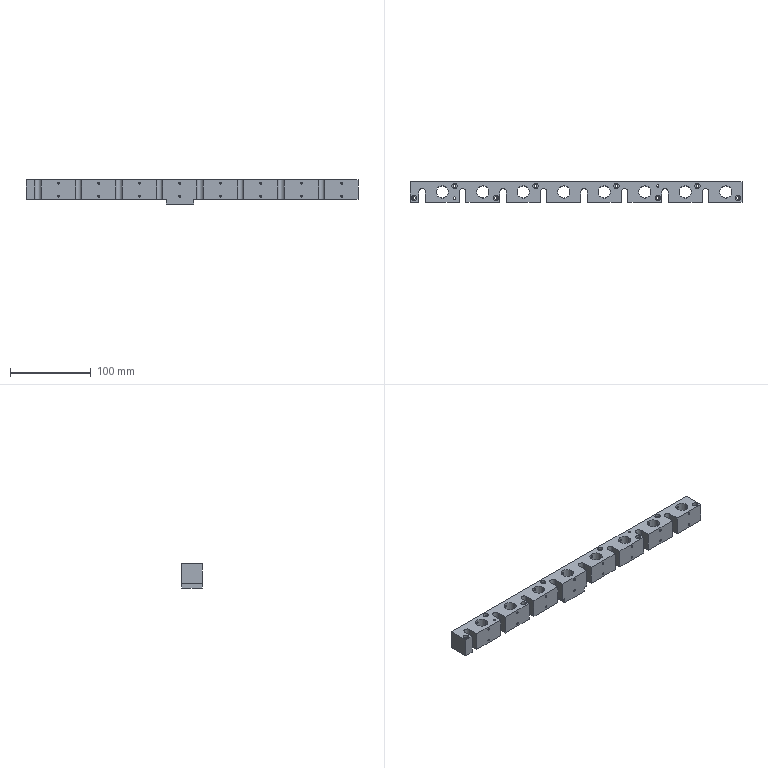Component | SolidWorks | 002MaterialPickingModuleA-1_004SidePlugModule-1_J-009-1 | 1 solid | 174 faces | box 410 x 25 x 30 mm | volume 188018 mm3 | cylinder 128 | plane 42 | cone 4 | commonest cylinder face diameters 2.5 x64 6.5 x16 3.4 x16 15 x16 8.1 x8 3 x4 3.3 x4 | material 45
build123d program:
from build123d import *

# Parameters (mm, degrees)
SKETCH1_W                                       = 440
SKETCH1_H                                       = 24
BOSS_EXTRUDE1_DEPTH                             = 12.5
SKETCH2_R                                       = 7.5
CUT_EXTRUDE1_DEPTH                              = 222.658
CUT_EXTRUDE2_DEPTH                              = 222.658
LPATTERN1_COUNT                                 = 8
LPATTERN1_PITCH                                 = 50
SKETCH4_W                                       = 34
SKETCH4_H                                       = 25
SKETCH4_R                                       = 7.5
BOSS_EXTRUDE2_DEPTH                             = 6
M4_TAPPED_HOLE1_D                               = 3.3
M4_TAPPED_HOLE1_DEPTH                           = 10.1
M4_TAPPED_HOLE1_TIP                             = 0.9914
SKETCH8_W                                       = 30
SKETCH8_H                                       = 25
CUT_EXTRUDE4_DEPTH                              = 223.388
M3_HEX_SOCKET_HEAD_CAP_SCREW_CBORE1_D           = 3.4
M3_HEX_SOCKET_HEAD_CAP_SCREW_CBORE1_CBORE_D     = 6.5
M3_HEX_SOCKET_HEAD_CAP_SCREW_CBORE1_CBORE_DEPTH = 3.4
SIZE_MM_DOWEL_PIN_HOLE1_D                       = 3
M3_TAPPED_HOLE1_D                               = 2.5
LPATTERN2_COUNT                                 = 8
LPATTERN2_PITCH                                 = 50


with BuildPart() as part:
    # Sketch1 → Boss-Extrude1 (new, symmetric)
    with BuildSketch(Plane(origin=(0, 0, 0), x_dir=(1, 0, 0), z_dir=(0, 1, 0))):
        Rectangle(SKETCH1_W, SKETCH1_H)
    extrude(amount=BOSS_EXTRUDE1_DEPTH, both=True)

    # Sketch2 → Cut-Extrude1 (cut, through all)
    with BuildSketch(Plane.XY.offset(12)):
        Circle(SKETCH2_R)
        with Locations((-50, 0)):
            Circle(SKETCH2_R)
        with Locations((-100, 0)):
            Circle(SKETCH2_R)
        with Locations((50, 0)):
            Circle(SKETCH2_R)
        with Locations((100, 0)):
            Circle(SKETCH2_R)
        with Locations((-150, 0)):
            Circle(SKETCH2_R)
        with Locations((150, 0)):
            Circle(SKETCH2_R)
        with Locations((-200, 0)):
            Circle(SKETCH2_R)
        with Locations((200, 0)):
            Circle(SKETCH2_R)
    extrude(amount=-CUT_EXTRUDE1_DEPTH, mode=Mode.SUBTRACT)

    # Sketch3 → Cut-Extrude2 (cut, through all)
    with BuildSketch(Plane.XY.offset(12)):
        with BuildLine():
            Line((-170.95, 0), (-170.95, -12.5))
            ThreePointArc((-170.95, -12.5), (-175, -16.55), (-179.05, -12.5))
            Line((-179.05, -12.5), (-179.05, 0))
            ThreePointArc((-179.05, 0), (-175, 4.05), (-170.95, 0))
        make_face()
    cut_extrude2 = extrude(amount=-CUT_EXTRUDE2_DEPTH, mode=Mode.SUBTRACT)

    # LPattern1: Cut-Extrude2 ×8
    with Locations(*[(i * LPATTERN1_PITCH, 0, 0) for i in range(1, LPATTERN1_COUNT)]):
        add(cut_extrude2, mode=Mode.SUBTRACT)

    # Sketch4 → Boss-Extrude2 (add)
    with BuildSketch(Plane(origin=(0, 0, -12), x_dir=(-1, 0, 0), z_dir=(0, 0, -1))):
        Rectangle(SKETCH4_W, SKETCH4_H)
        with Locations(Location((0, 0, 0), (0, 0, 180))):
            Circle(SKETCH4_R, mode=Mode.SUBTRACT)
    extrude(amount=BOSS_EXTRUDE2_DEPTH)

    # M4 Tapped Hole1
    with Locations(Plane(origin=(0, 12.5, 0), x_dir=(1, 0, 0), z_dir=(0, 1, 0))):
        with Locations((12.5, 13), (12.5, -6)):
            Hole(M4_TAPPED_HOLE1_D / 2, depth=M4_TAPPED_HOLE1_DEPTH)
            with Locations((0, 0, -(M4_TAPPED_HOLE1_DEPTH + M4_TAPPED_HOLE1_TIP / 2))):  # 118° drill point
                Cone(0, M4_TAPPED_HOLE1_D / 2, M4_TAPPED_HOLE1_TIP, mode=Mode.SUBTRACT)

    # Sketch8 → Cut-Extrude4 (cut, through all)
    with BuildSketch(Plane.XY.offset(12)):
        with Locations((-205, 0)):
            Rectangle(SKETCH8_W, SKETCH8_H)
    extrude(amount=-CUT_EXTRUDE4_DEPTH, mode=Mode.SUBTRACT)

    # M3 Hex Socket Head Cap Screw CBORE1 (through all)
    with Locations(Plane.XY.offset(12)):
        with Locations((-35, 7.5), (65, 7.5), (-84.05, -7.5), (-135, 7.5), (-185, -7.5), (115.95, -7.5), (165, 7.5), (215, -7.5)):
            CounterBoreHole(M3_HEX_SOCKET_HEAD_CAP_SCREW_CBORE1_D / 2, M3_HEX_SOCKET_HEAD_CAP_SCREW_CBORE1_CBORE_D / 2, M3_HEX_SOCKET_HEAD_CAP_SCREW_CBORE1_CBORE_DEPTH)

    # Size mm Dowel Pin Hole1 (through all)
    with Locations(Plane.XY.offset(12)):
        with Locations((-135, -7.5), (115.95, 7.5)):
            Hole(SIZE_MM_DOWEL_PIN_HOLE1_D / 2)

    # M3 Tapped Hole1 (through all)
    with Locations(Plane(origin=(0, 12.5, 0), x_dir=(1, 0, 0), z_dir=(0, 1, 0))):
        with Locations((200, 8), (200, -8)):
            m3_tapped_hole1 = Hole(M3_TAPPED_HOLE1_D / 2)

    # LPattern2: M3 Tapped Hole1 ×8
    with Locations(*[(-i * LPATTERN2_PITCH, 0, 0) for i in range(1, LPATTERN2_COUNT)]):
        add(m3_tapped_hole1, mode=Mode.SUBTRACT)


solid = part.part

# Placed as in the assembly
solid = solid.moved(Location((220.324, 296.019, 440.231), (0, 0, 0)))